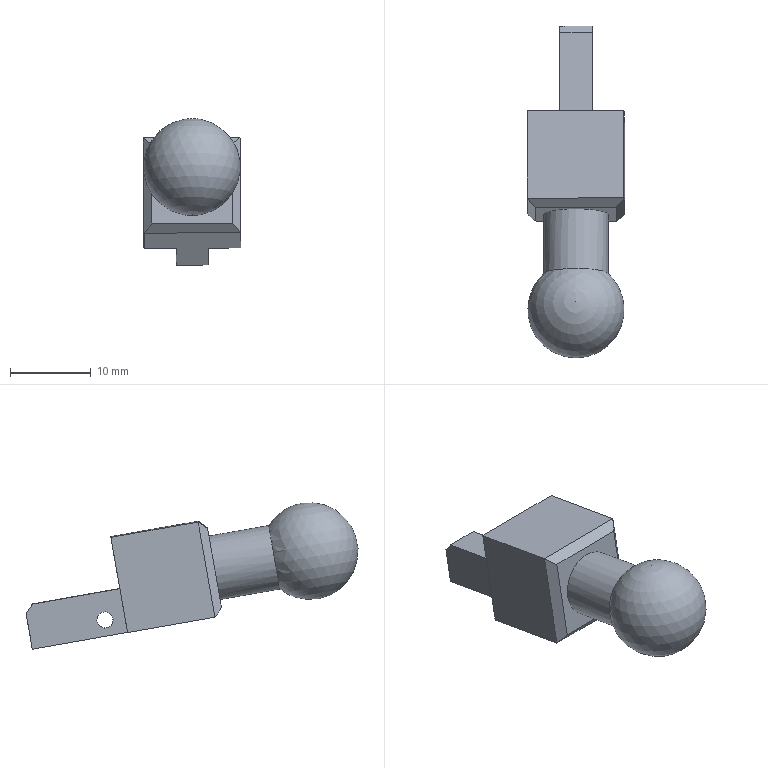Component | NX | BALL_JOINT_BASE | 1 solid | 20 faces | volume 3185 mm3 | plane 15 | cylinder 3 | sphere 1 | cone 1 | commonest cylinder face diameters 8 x1 2 x1 3.5 x1